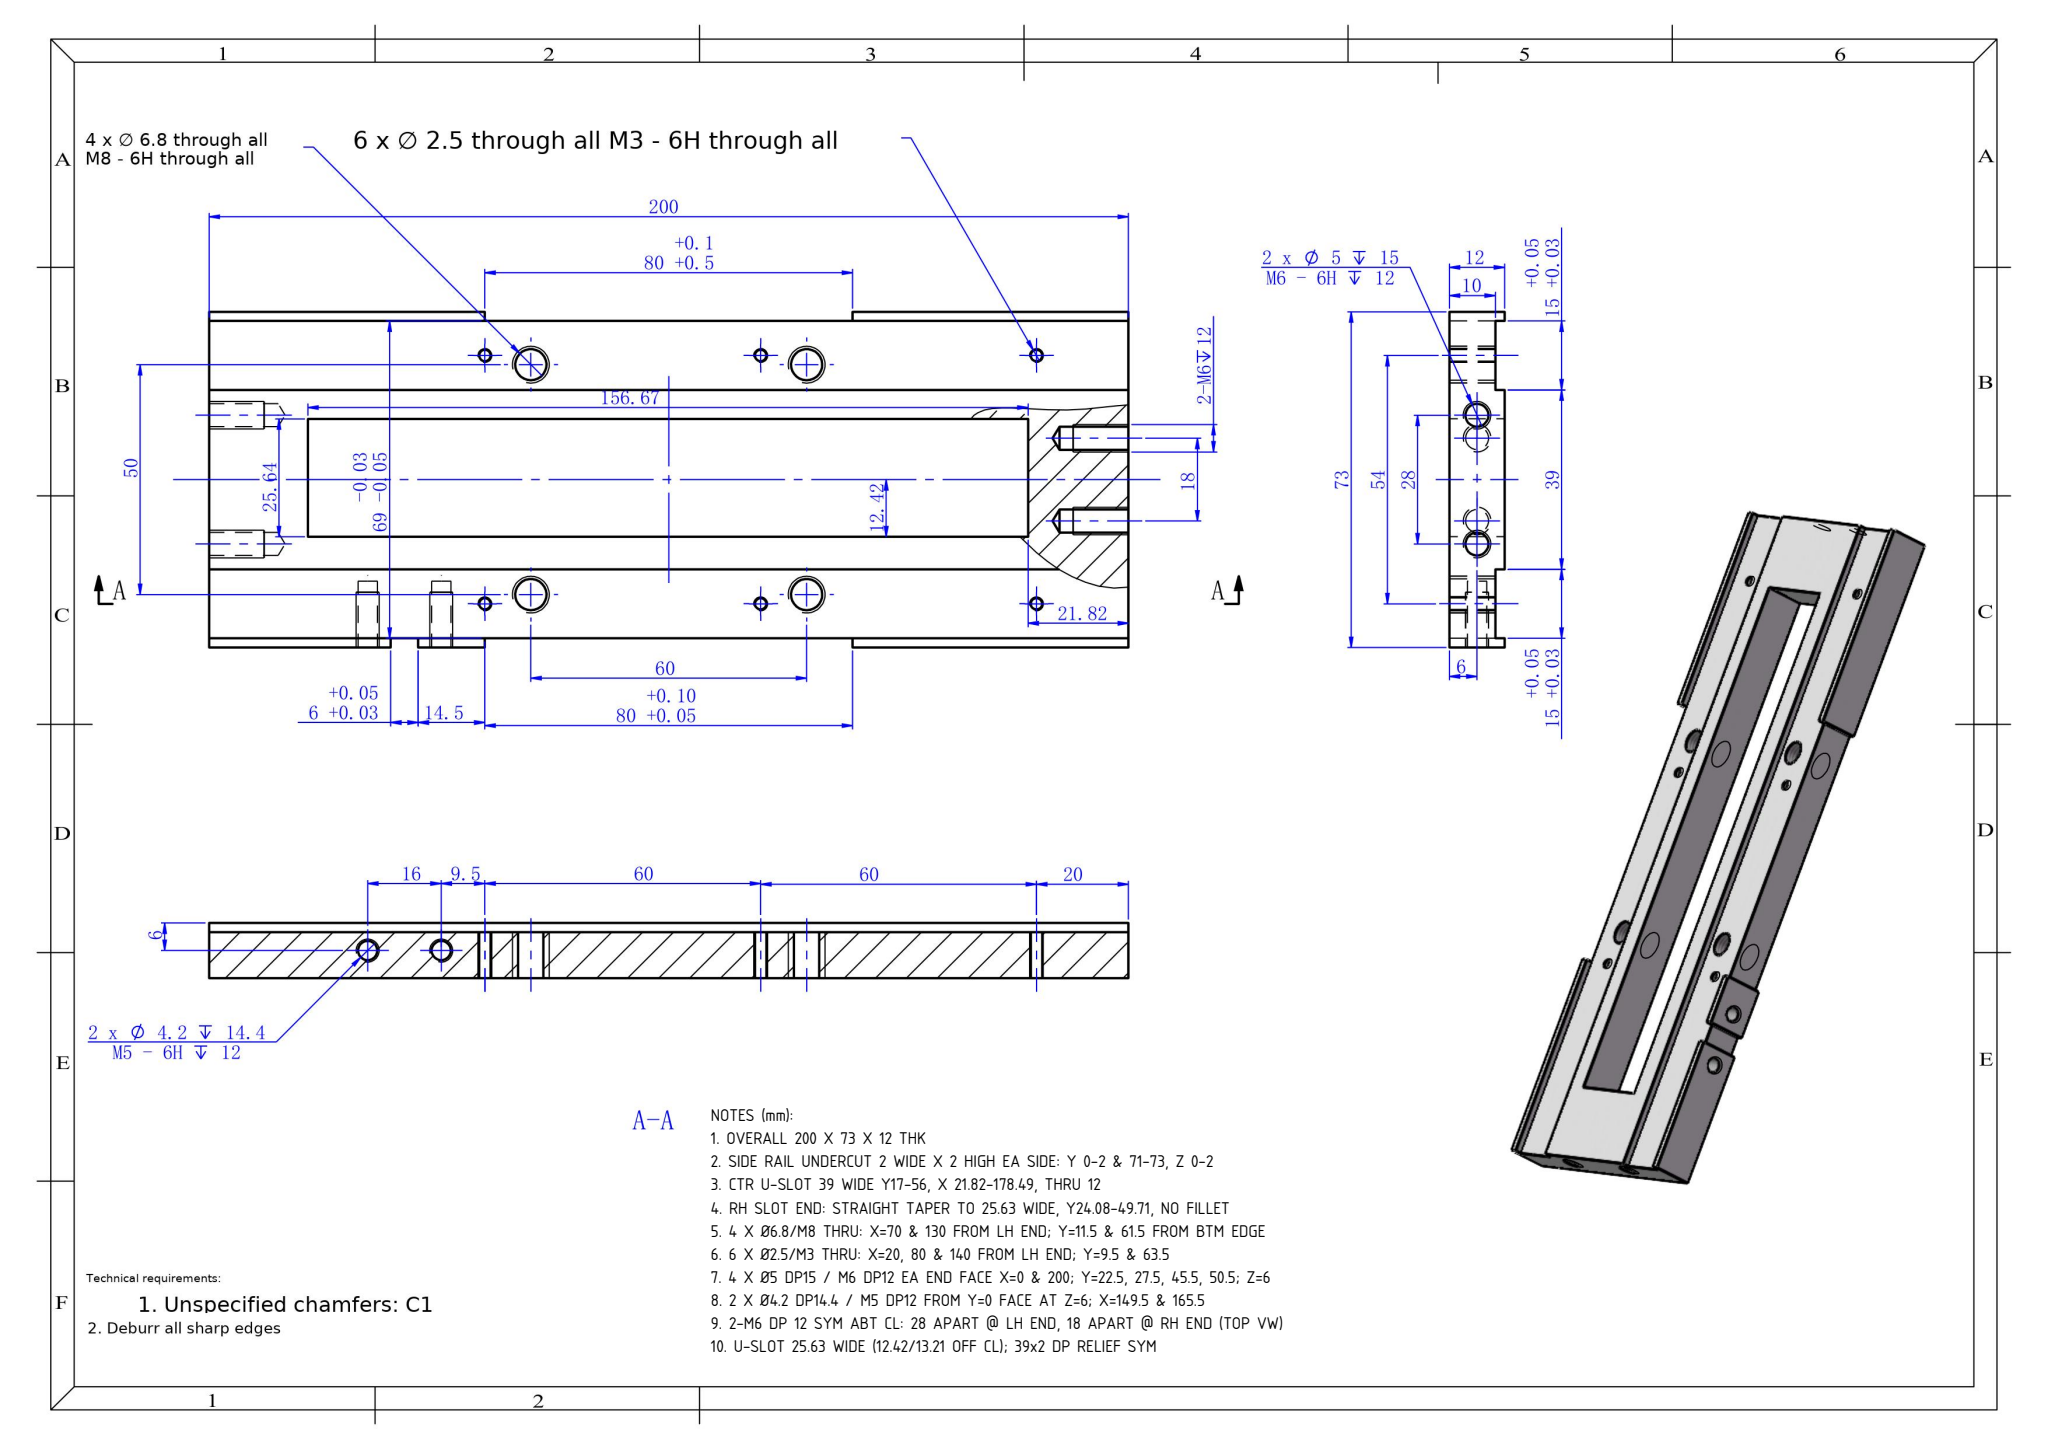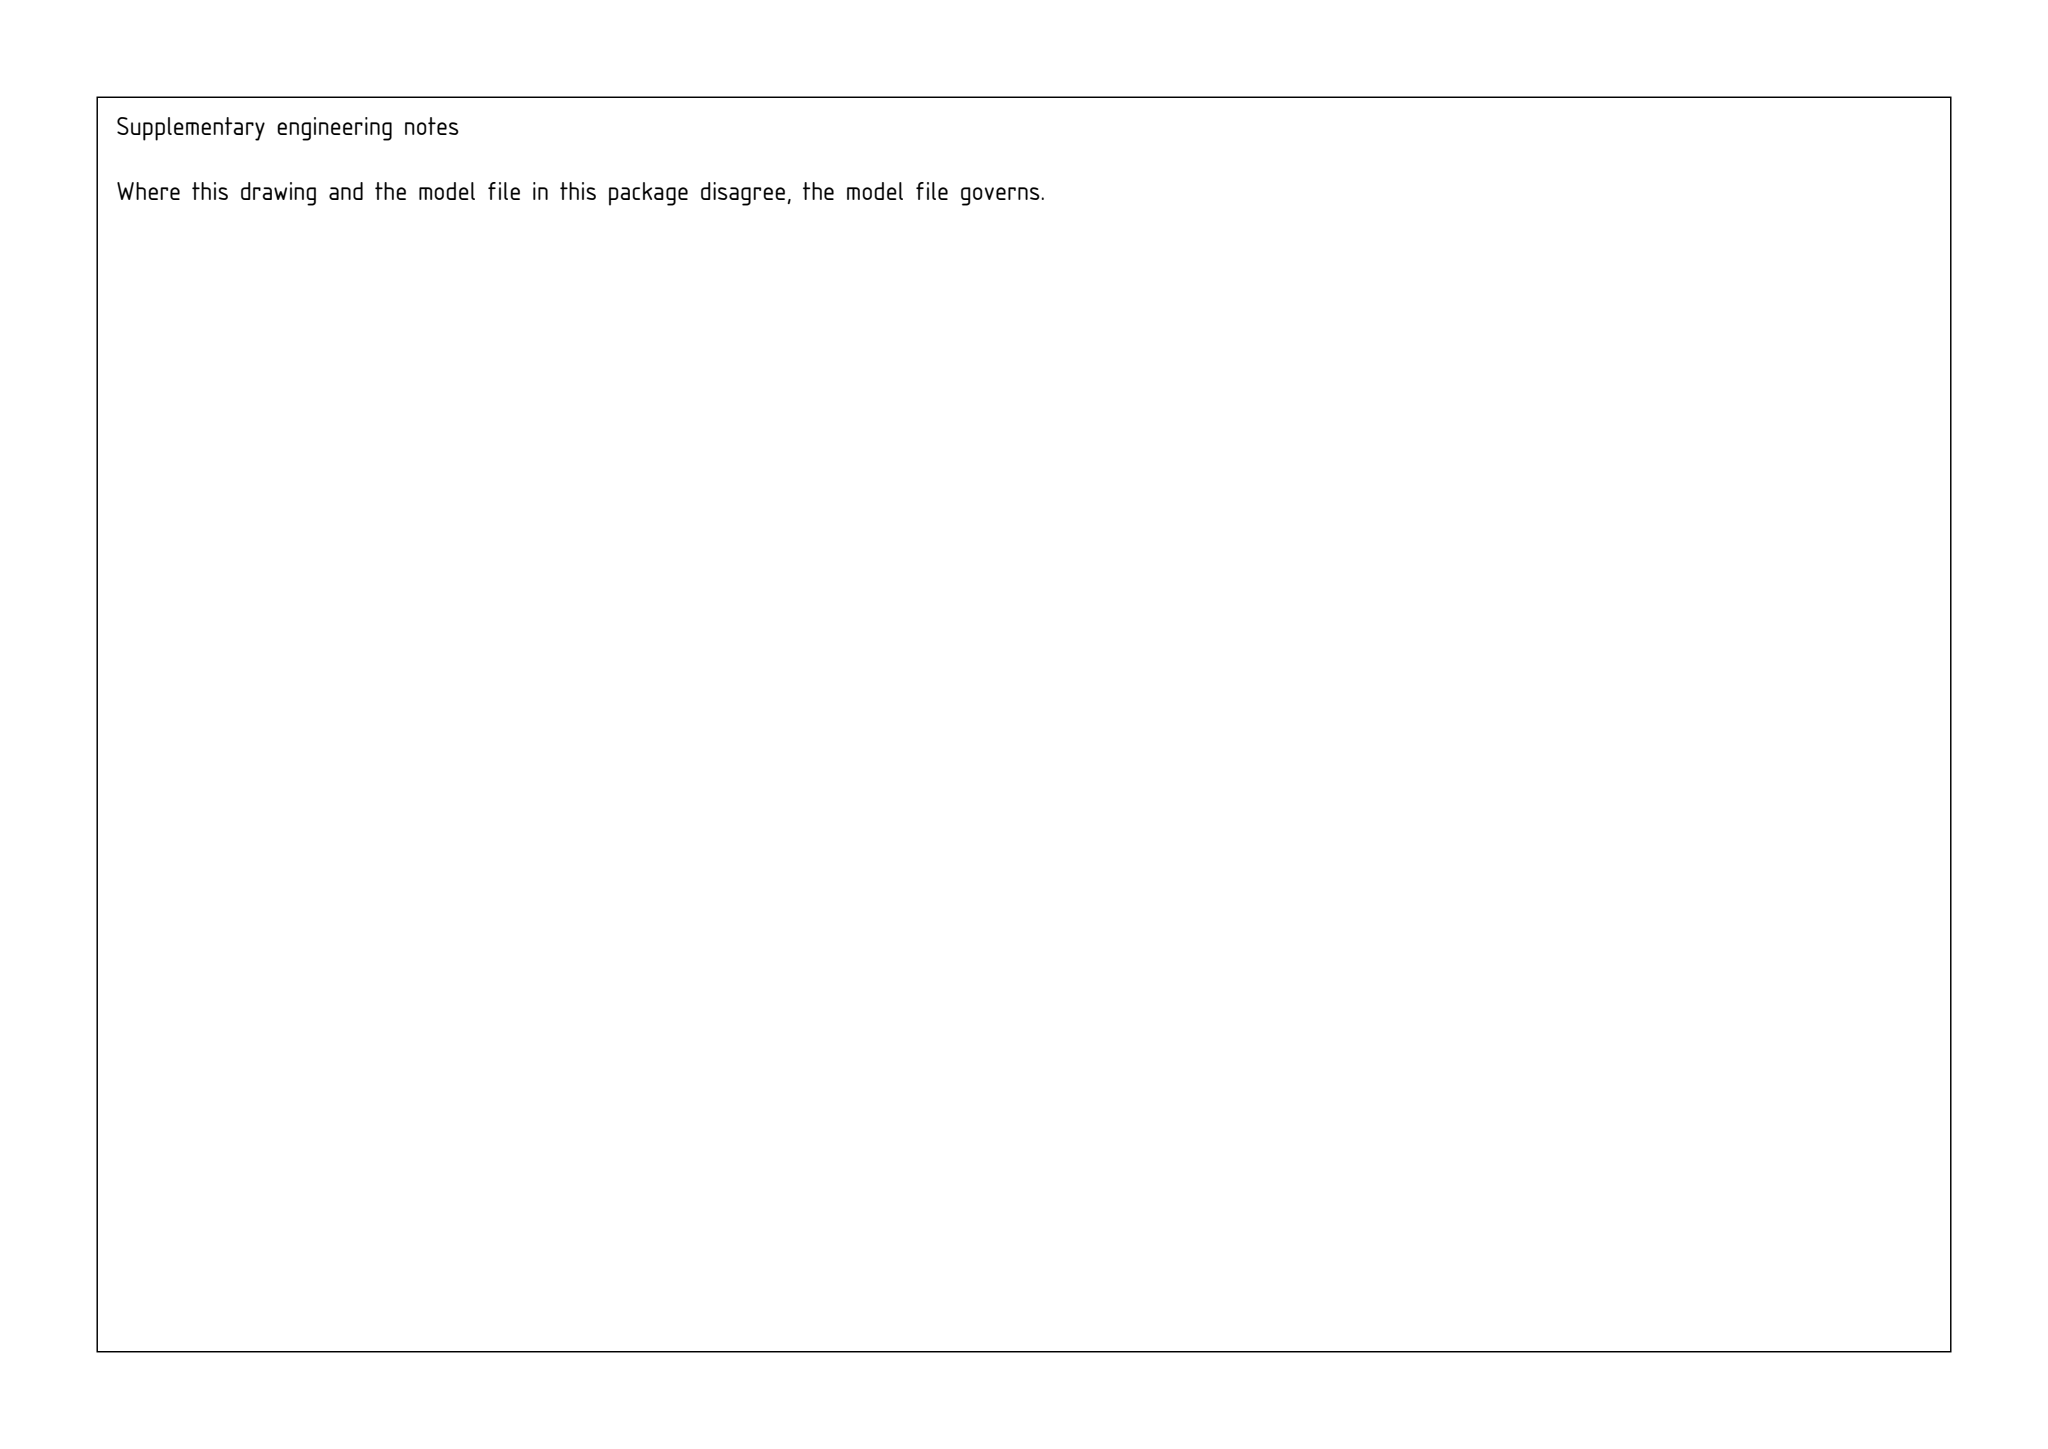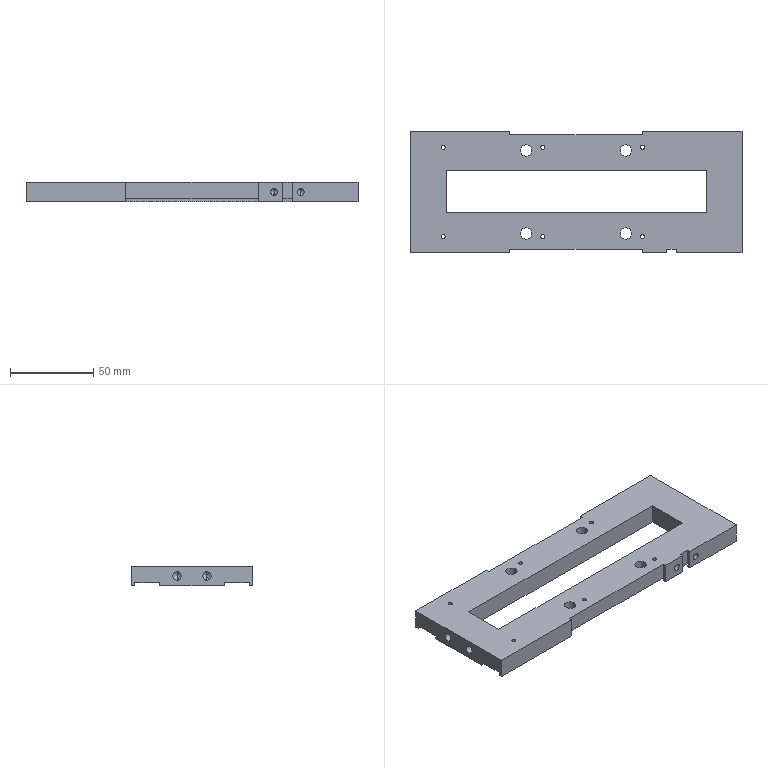Part | SolidWorks | mm | 1 solid | 80 faces | box 200 x 73 x 12 mm | volume 107641 mm3 | plane 36 | cylinder 32 | cone 12 | commonest cylinder face diameters 2.5 x12 6.8 x8 5 x8 4.2 x4
Drawing notes:
OVERALL 200 X 73 X 12 THK | from the solid: bbox_xyz 200,73,12
SIDE RAIL UNDERCUT 2 WIDE X 2 HIGH EA SIDE: Y 0-2 & 71-73, Z 0-2 | from the solid: y planes 2 & 71 with z plane 2; bbox Y=73, Z=12
CTR U-SLOT 39 WIDE Y17-56, X 21.82-178.49, THRU 12 | from the solid: x planes 21.82 & 178.49 (=156.67); y planes 17 & 56; z 0-12
RH SLOT END: STRAIGHT TAPER TO 25.63 WIDE, Y24.08-49.71, NO FILLET | from the solid: y planes 24.08 & 49.71 (25.63 wide); fillet_radii empty
4 X Ø6.8/M8 THRU: X=70 & 130 FROM LH END; Y=11.5 & 61.5 FROM BTM EDGE | from the solid: cyl Ø6.8 z-axis at (70,11.5),(70,61.5),(130,11.5),(130,61.5)
6 X Ø2.5/M3 THRU: X=20, 80 & 140 FROM LH END; Y=9.5 & 63.5 | from the solid: cyl Ø2.5 z-axis at x=20,80,140 with y=9.5 and 63.5, thru 12 plate
4 X Ø5 DP15 / M6 DP12 EA END FACE X=0 & 200; Y=22.5, 27.5, 45.5, 50.5; Z=6 | from the solid: cyl Ø5 x-axis L=15 at y=22.5,27.5,45.5,50.5, z=6, count 2 each
2 X Ø4.2 DP14.4 / M5 DP12 FROM Y=0 FACE AT Z=6; X=149.5 & 165.5 | from the solid: cyl Ø4.2 y-axis at x=149.5 & 165.5, z=6, L=14.4
2-M6 DP 12 SYM ABT CL: 28 APART @ LH END, 18 APART @ RH END (TOP VW) | from the solid: Ø5 x-axis holes: x=185-200 end at Y22.5 & 50.5 (28 apart, ±14 from Y CL 36.5); x=0-15 end at Y27.5 & 45.5 (18 apart, ±9 from CL). LH end of top view = model x=200 end (M5 Ø4.2 holes at x=149.5/165.5 appear at left).
U-SLOT 25.63 WIDE (12.42/13.21 OFF CL); 39x2 DP RELIEF SYM | from the solid: Slot walls y=24.08 & 49.71 over x=21.8-178.5, full 12 thk (width 25.63; CL of 73 = 36.5 → 12.42 and 13.21). Separate z=0 face y17-56 full length = 39 wide x 2 deep relief, sym abt CL.
build123d program:
from build123d import *

# Parameters (mm, degrees)
SKETCH1_W             = 200
SKETCH1_H             = 73
BOSS_EXTRUDE1_DEPTH   = 12
SKETCH2_W             = 2
SKETCH2_H             = 15
CUT_EXTRUDE1_DEPTH    = 217.905
SKETCH3_W             = 6
SKETCH3_H             = 2
CUT_EXTRUDE2_DEPTH    = 167.759
M5_TAPPED_HOLE1_D     = 4.2
M5_TAPPED_HOLE1_DEPTH = 14.4
M5_TAPPED_HOLE1_TIP   = 1.262
M6_TAPPED_HOLE1_D     = 5
M6_TAPPED_HOLE1_DEPTH = 15
M6_TAPPED_HOLE1_TIP   = 1.502
M6_TAPPED_HOLE2_D     = 5
M6_TAPPED_HOLE2_DEPTH = 15
M6_TAPPED_HOLE2_TIP   = 1.502
M8_TAPPED_HOLE1_D     = 6.8
SKETCH12_W            = 80
SKETCH12_H            = 2
CUT_EXTRUDE3_DEPTH    = 167.759
M3_TAPPED_HOLE1_D     = 2.5
SKETCH15_W            = 156.672
SKETCH15_H            = 25.637
CUT_EXTRUDE4_DEPTH    = 32


with BuildPart() as part:
    # Sketch1 → Boss-Extrude1 (new body)
    with BuildSketch(Plane.XY):
        with Locations((-44.086, 46.59)):
            Rectangle(SKETCH1_W, SKETCH1_H)
    extrude(amount=BOSS_EXTRUDE1_DEPTH)

    # Sketch2 → Cut-Extrude1 (cut, through all)
    with BuildSketch(Plane(origin=(55.914, 0, 0), x_dir=(0, 0, -1), z_dir=(1, 0, 0))):
        with Locations((-1, 19.59)):
            Rectangle(SKETCH2_W, SKETCH2_H)
        with Locations((-1, 73.59)):
            Rectangle(SKETCH2_W, SKETCH2_H)
    extrude(amount=-CUT_EXTRUDE1_DEPTH, mode=Mode.SUBTRACT)

    # Sketch3 → Cut-Extrude2 (cut, through all)
    with BuildSketch(Plane.XY.offset(12)):
        with Locations((13.414, 11.09)):
            Rectangle(SKETCH3_W, SKETCH3_H)
    extrude(amount=-CUT_EXTRUDE2_DEPTH, mode=Mode.SUBTRACT)

    # M5 Tapped Hole1
    with Locations(Plane(origin=(0, 10.09, 0), x_dir=(-1, 0, 0), z_dir=(0, -1, 0))):
        with Locations((-5.414, -6), (-21.414, -6)):
            Hole(M5_TAPPED_HOLE1_D / 2, depth=M5_TAPPED_HOLE1_DEPTH)
            with Locations((0, 0, -(M5_TAPPED_HOLE1_DEPTH + M5_TAPPED_HOLE1_TIP / 2))):  # 118° drill point
                Cone(0, M5_TAPPED_HOLE1_D / 2, M5_TAPPED_HOLE1_TIP, mode=Mode.SUBTRACT)

    # M6 Tapped Hole1
    with Locations(Plane(origin=(55.914, 0, 0), x_dir=(0, 0, -1), z_dir=(1, 0, 0))):
        with Locations((-6, 60.59), (-6, 32.59)):
            Hole(M6_TAPPED_HOLE1_D / 2, depth=M6_TAPPED_HOLE1_DEPTH)
            with Locations((0, 0, -(M6_TAPPED_HOLE1_DEPTH + M6_TAPPED_HOLE1_TIP / 2))):  # 118° drill point
                Cone(0, M6_TAPPED_HOLE1_D / 2, M6_TAPPED_HOLE1_TIP, mode=Mode.SUBTRACT)

    # M6 Tapped Hole2
    with Locations(Plane.ZY.offset(144.086)):
        with Locations((6, 37.59), (6, 55.59)):
            Hole(M6_TAPPED_HOLE2_D / 2, depth=M6_TAPPED_HOLE2_DEPTH)
            with Locations((0, 0, -(M6_TAPPED_HOLE2_DEPTH + M6_TAPPED_HOLE2_TIP / 2))):  # 118° drill point
                Cone(0, M6_TAPPED_HOLE2_D / 2, M6_TAPPED_HOLE2_TIP, mode=Mode.SUBTRACT)

    # M8 Tapped Hole1 (through all)
    with Locations(Plane.XY.offset(12)):
        with Locations((-14.086, 21.59), (-74.086, 21.59), (-74.086, 71.59), (-14.086, 71.59)):
            Hole(M8_TAPPED_HOLE1_D / 2)

    # Sketch12 → Cut-Extrude3 (cut, through all)
    with BuildSketch(Plane.XY.offset(12)):
        with Locations((-44.086, 82.09)):
            Rectangle(SKETCH12_W, SKETCH12_H)
        with Locations((-44.086, 11.09)):
            Rectangle(SKETCH12_W, SKETCH12_H)
    extrude(amount=-CUT_EXTRUDE3_DEPTH, mode=Mode.SUBTRACT)

    # M3 Tapped Hole1 (through all)
    with Locations(Plane(origin=(0, 0, 2), x_dir=(-1, 0, 0), z_dir=(0, 0, -1))):
        with Locations((124.086, 19.59), (64.086, 19.59), (4.086, 19.59), (4.086, 73.59), (64.086, 73.59), (124.086, 73.59)):
            Hole(M3_TAPPED_HOLE1_D / 2)

    # Sketch15 → Cut-Extrude4 (cut)
    with BuildSketch(Plane(origin=(0, 0, 0), x_dir=(-1, 0, 0), z_dir=(0, 0, -1))):
        with Locations((43.928, 46.986)):
            Rectangle(SKETCH15_W, SKETCH15_H)
    extrude(amount=-CUT_EXTRUDE4_DEPTH, mode=Mode.SUBTRACT)


solid = part.part